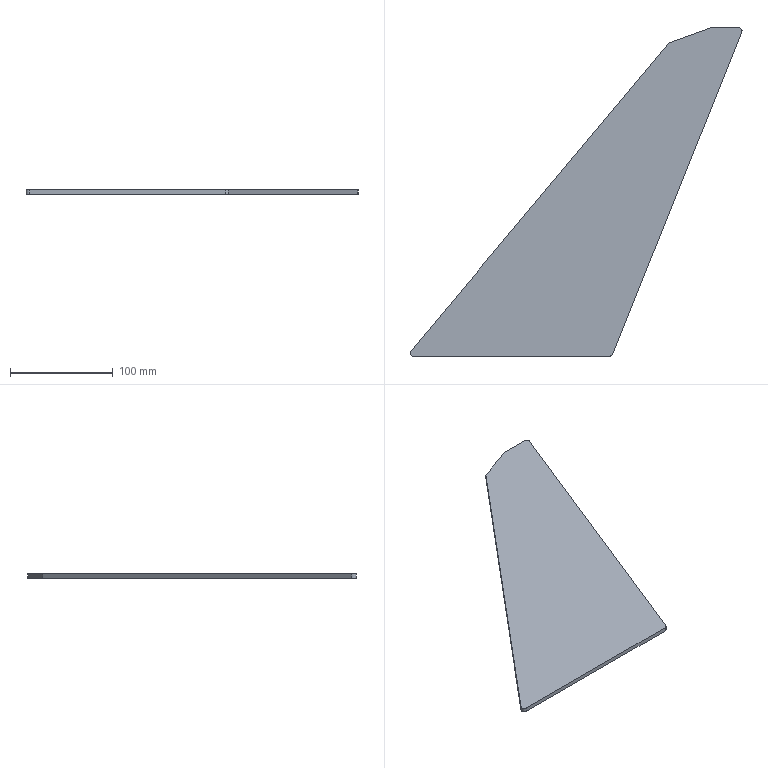Component | SolidWorks | 03-01MotorBracket1-1 | 1 solid | 11 faces | box 323.64 x 320 x 4 mm | volume 165534 mm3 | plane 7 | cylinder 4 | commonest cylinder face diameters 6 x4
STEP:
#1=COLOUR_RGB('',0.7922,0.8196,0.9333);
#2=FILL_AREA_STYLE_COLOUR('',#1);
#3=FILL_AREA_STYLE('',(#2));
#4=SURFACE_STYLE_FILL_AREA(#3);
#5=SURFACE_SIDE_STYLE('',(#4));
#6=SURFACE_STYLE_USAGE(.BOTH.,#5);
#7=PRESENTATION_STYLE_ASSIGNMENT((#6));
#8=CARTESIAN_POINT('',(11.927,12.48,14.961));
#9=VERTEX_POINT('',#8);
#10=CARTESIAN_POINT('',(11.918,12.436,14.961));
#11=VERTEX_POINT('',#10);
#12=CARTESIAN_POINT('',(11.809,12.48,14.961));
#13=DIRECTION('',(0.,0.,-1.));
#14=DIRECTION('',(1.,0.,0.));
#15=AXIS2_PLACEMENT_3D('',#12,#13,#14);
#16=CIRCLE('',#15,0.1181);
#17=EDGE_CURVE('',#9,#11,#16,.T.);
#18=ORIENTED_EDGE('',*,*,#17,.F.);
#19=CARTESIAN_POINT('',(11.927,12.48,15.118));
#20=VERTEX_POINT('',#19);
#21=CARTESIAN_POINT('',(11.927,12.48,14.961));
#22=DIRECTION('',(0.,0.,1.));
#23=VECTOR('',#22,39.37);
#24=LINE('',#21,#23);
#25=EDGE_CURVE('',#9,#20,#24,.T.);
#26=ORIENTED_EDGE('',*,*,#25,.T.);
#27=CARTESIAN_POINT('',(11.918,12.436,15.118));
#28=VERTEX_POINT('',#27);
#29=CARTESIAN_POINT('',(11.809,12.48,15.118));
#30=DIRECTION('',(0.,0.,1.));
#31=DIRECTION('',(1.,0.,0.));
#32=AXIS2_PLACEMENT_3D('',#29,#30,#31);
#33=CIRCLE('',#32,0.1181);
#34=EDGE_CURVE('',#28,#20,#33,.T.);
#35=ORIENTED_EDGE('',*,*,#34,.F.);
#36=CARTESIAN_POINT('',(11.918,12.436,14.961));
#37=DIRECTION('',(0.,0.,1.));
#38=VECTOR('',#37,39.37);
#39=LINE('',#36,#38);
#40=EDGE_CURVE('',#11,#28,#39,.T.);
#41=ORIENTED_EDGE('',*,*,#40,.F.);
#42=EDGE_LOOP('',(#18,#26,#35,#41));
#43=FACE_OUTER_BOUND('',#42,.T.);
#44=CARTESIAN_POINT('',(11.809,12.48,14.961));
#45=DIRECTION('',(0.,0.,1.));
#46=DIRECTION('',(1.,0.,0.));
#47=AXIS2_PLACEMENT_3D('',#44,#45,#46);
#48=CYLINDRICAL_SURFACE('',#47,0.1181);
#49=ADVANCED_FACE('',(#43),#48,.T.);
#50=CARTESIAN_POINT('',(9.14,12.025,15.118));
#51=VERTEX_POINT('',#50);
#52=CARTESIAN_POINT('',(-0.7874,0.194,15.118));
#53=VERTEX_POINT('',#52);
#54=CARTESIAN_POINT('',(9.621,12.598,15.118));
#55=DIRECTION('',(-0.6428,-0.766,0.));
#56=VECTOR('',#55,39.37);
#57=LINE('',#54,#56);
#58=EDGE_CURVE('',#51,#53,#57,.T.);
#59=ORIENTED_EDGE('',*,*,#58,.F.);
#60=CARTESIAN_POINT('',(9.14,12.025,14.961));
#61=VERTEX_POINT('',#60);
#62=CARTESIAN_POINT('',(9.14,12.025,14.724));
#63=DIRECTION('',(0.,0.,1.));
#64=VECTOR('',#63,39.37);
#65=LINE('',#62,#64);
#66=EDGE_CURVE('',#61,#51,#65,.T.);
#67=ORIENTED_EDGE('',*,*,#66,.F.);
#68=CARTESIAN_POINT('',(-0.7874,0.194,14.961));
#69=VERTEX_POINT('',#68);
#70=CARTESIAN_POINT('',(9.621,12.598,14.961));
#71=DIRECTION('',(-0.6428,-0.766,0.));
#72=VECTOR('',#71,39.37);
#73=LINE('',#70,#72);
#74=EDGE_CURVE('',#61,#69,#73,.T.);
#75=ORIENTED_EDGE('',*,*,#74,.T.);
#76=CARTESIAN_POINT('',(-0.7874,0.194,14.961));
#77=DIRECTION('',(0.,0.,1.));
#78=VECTOR('',#77,39.37);
#79=LINE('',#76,#78);
#80=EDGE_CURVE('',#69,#53,#79,.T.);
#81=ORIENTED_EDGE('',*,*,#80,.T.);
#82=EDGE_LOOP('',(#59,#67,#75,#81));
#83=FACE_OUTER_BOUND('',#82,.T.);
#84=CARTESIAN_POINT('',(9.621,12.598,14.961));
#85=DIRECTION('',(-0.766,0.6428,0.));
#86=DIRECTION('',(-0.6428,-0.766,0.));
#87=AXIS2_PLACEMENT_3D('',#84,#85,#86);
#88=PLANE('',#87);
#89=ADVANCED_FACE('',(#83),#88,.T.);
#90=CARTESIAN_POINT('',(11.809,12.598,14.961));
#91=VERTEX_POINT('',#90);
#92=CARTESIAN_POINT('',(10.715,12.598,14.961));
#93=VERTEX_POINT('',#92);
#94=CARTESIAN_POINT('',(11.983,12.598,14.961));
#95=DIRECTION('',(-1.,-0.,0.));
#96=VECTOR('',#95,39.37);
#97=LINE('',#94,#96);
#98=EDGE_CURVE('',#91,#93,#97,.T.);
#99=ORIENTED_EDGE('',*,*,#98,.T.);
#100=CARTESIAN_POINT('',(10.715,12.598,15.118));
#101=VERTEX_POINT('',#100);
#102=CARTESIAN_POINT('',(10.715,12.598,14.724));
#103=DIRECTION('',(0.,0.,1.));
#104=VECTOR('',#103,39.37);
#105=LINE('',#102,#104);
#106=EDGE_CURVE('',#93,#101,#105,.T.);
#107=ORIENTED_EDGE('',*,*,#106,.T.);
#108=CARTESIAN_POINT('',(11.809,12.598,15.118));
#109=VERTEX_POINT('',#108);
#110=CARTESIAN_POINT('',(11.983,12.598,15.118));
#111=DIRECTION('',(-1.,-0.,0.));
#112=VECTOR('',#111,39.37);
#113=LINE('',#110,#112);
#114=EDGE_CURVE('',#109,#101,#113,.T.);
#115=ORIENTED_EDGE('',*,*,#114,.F.);
#116=CARTESIAN_POINT('',(11.809,12.598,14.961));
#117=DIRECTION('',(0.,0.,-1.));
#118=VECTOR('',#117,39.37);
#119=LINE('',#116,#118);
#120=EDGE_CURVE('',#109,#91,#119,.T.);
#121=ORIENTED_EDGE('',*,*,#120,.T.);
#122=EDGE_LOOP('',(#99,#107,#115,#121));
#123=FACE_OUTER_BOUND('',#122,.T.);
#124=CARTESIAN_POINT('',(11.983,12.598,14.961));
#125=DIRECTION('',(-0.,1.,0.));
#126=DIRECTION('',(-1.,-0.,0.));
#127=AXIS2_PLACEMENT_3D('',#124,#125,#126);
#128=PLANE('',#127);
#129=ADVANCED_FACE('',(#123),#128,.T.);
#130=CARTESIAN_POINT('',(-3.635,7.376,14.961));
#131=DIRECTION('',(-0.9397,-0.342,0.));
#132=VECTOR('',#131,39.37);
#133=LINE('',#130,#132);
#134=EDGE_CURVE('',#93,#61,#133,.T.);
#135=ORIENTED_EDGE('',*,*,#134,.F.);
#136=ORIENTED_EDGE('',*,*,#98,.F.);
#137=CARTESIAN_POINT('',(11.809,12.48,14.961));
#138=DIRECTION('',(0.,0.,-1.));
#139=DIRECTION('',(1.,0.,0.));
#140=AXIS2_PLACEMENT_3D('',#137,#138,#139);
#141=CIRCLE('',#140,0.1181);
#142=EDGE_CURVE('',#91,#9,#141,.T.);
#143=ORIENTED_EDGE('',*,*,#142,.T.);
#144=ORIENTED_EDGE('',*,*,#17,.T.);
#145=CARTESIAN_POINT('',(6.954,0.07409,14.961));
#146=VERTEX_POINT('',#145);
#147=CARTESIAN_POINT('',(6.924,-0.,14.961));
#148=DIRECTION('',(0.3727,0.928,0.));
#149=VECTOR('',#148,39.37);
#150=LINE('',#147,#149);
#151=EDGE_CURVE('',#146,#11,#150,.T.);
#152=ORIENTED_EDGE('',*,*,#151,.F.);
#153=CARTESIAN_POINT('',(6.844,-0.,14.961));
#154=VERTEX_POINT('',#153);
#155=CARTESIAN_POINT('',(6.844,0.1181,14.961));
#156=DIRECTION('',(0.,0.,-1.));
#157=DIRECTION('',(1.,-0.,0.));
#158=AXIS2_PLACEMENT_3D('',#155,#156,#157);
#159=CIRCLE('',#158,0.1181);
#160=EDGE_CURVE('',#146,#154,#159,.T.);
#161=ORIENTED_EDGE('',*,*,#160,.T.);
#162=CARTESIAN_POINT('',(-0.6969,-0.,14.961));
#163=VERTEX_POINT('',#162);
#164=CARTESIAN_POINT('',(-0.9502,-0.,14.961));
#165=DIRECTION('',(1.,0.,0.));
#166=VECTOR('',#165,39.37);
#167=LINE('',#164,#166);
#168=EDGE_CURVE('',#163,#154,#167,.T.);
#169=ORIENTED_EDGE('',*,*,#168,.F.);
#170=CARTESIAN_POINT('',(-0.6969,0.1181,14.961));
#171=DIRECTION('',(0.,0.,-1.));
#172=DIRECTION('',(1.,0.,0.));
#173=AXIS2_PLACEMENT_3D('',#170,#171,#172);
#174=CIRCLE('',#173,0.1181);
#175=EDGE_CURVE('',#163,#69,#174,.T.);
#176=ORIENTED_EDGE('',*,*,#175,.T.);
#177=ORIENTED_EDGE('',*,*,#74,.F.);
#178=EDGE_LOOP('',(#135,#136,#143,#144,#152,#161,#169,#176,#177));
#179=FACE_OUTER_BOUND('',#178,.T.);
#180=CARTESIAN_POINT('',(-0.9502,-0.,14.961));
#181=DIRECTION('',(0.,0.,1.));
#182=DIRECTION('',(1.,0.,0.));
#183=AXIS2_PLACEMENT_3D('',#180,#181,#182);
#184=PLANE('',#183);
#185=ADVANCED_FACE('',(#179),#184,.F.);
#186=ORIENTED_EDGE('',*,*,#114,.T.);
#187=CARTESIAN_POINT('',(-3.635,7.376,15.118));
#188=DIRECTION('',(-0.9397,-0.342,0.));
#189=VECTOR('',#188,39.37);
#190=LINE('',#187,#189);
#191=EDGE_CURVE('',#101,#51,#190,.T.);
#192=ORIENTED_EDGE('',*,*,#191,.T.);
#193=ORIENTED_EDGE('',*,*,#58,.T.);
#194=CARTESIAN_POINT('',(-0.6969,-0.,15.118));
#195=VERTEX_POINT('',#194);
#196=CARTESIAN_POINT('',(-0.6969,0.1181,15.118));
#197=DIRECTION('',(0.,0.,1.));
#198=DIRECTION('',(1.,0.,0.));
#199=AXIS2_PLACEMENT_3D('',#196,#197,#198);
#200=CIRCLE('',#199,0.1181);
#201=EDGE_CURVE('',#53,#195,#200,.T.);
#202=ORIENTED_EDGE('',*,*,#201,.T.);
#203=CARTESIAN_POINT('',(6.844,-0.,15.118));
#204=VERTEX_POINT('',#203);
#205=CARTESIAN_POINT('',(-0.9502,-0.,15.118));
#206=DIRECTION('',(1.,0.,0.));
#207=VECTOR('',#206,39.37);
#208=LINE('',#205,#207);
#209=EDGE_CURVE('',#195,#204,#208,.T.);
#210=ORIENTED_EDGE('',*,*,#209,.T.);
#211=CARTESIAN_POINT('',(6.954,0.07409,15.118));
#212=VERTEX_POINT('',#211);
#213=CARTESIAN_POINT('',(6.844,0.1181,15.118));
#214=DIRECTION('',(0.,0.,1.));
#215=DIRECTION('',(1.,0.,0.));
#216=AXIS2_PLACEMENT_3D('',#213,#214,#215);
#217=CIRCLE('',#216,0.1181);
#218=EDGE_CURVE('',#204,#212,#217,.T.);
#219=ORIENTED_EDGE('',*,*,#218,.T.);
#220=CARTESIAN_POINT('',(6.924,-0.,15.118));
#221=DIRECTION('',(0.3727,0.928,0.));
#222=VECTOR('',#221,39.37);
#223=LINE('',#220,#222);
#224=EDGE_CURVE('',#212,#28,#223,.T.);
#225=ORIENTED_EDGE('',*,*,#224,.T.);
#226=ORIENTED_EDGE('',*,*,#34,.T.);
#227=CARTESIAN_POINT('',(11.809,12.48,15.118));
#228=DIRECTION('',(0.,0.,1.));
#229=DIRECTION('',(1.,0.,0.));
#230=AXIS2_PLACEMENT_3D('',#227,#228,#229);
#231=CIRCLE('',#230,0.1181);
#232=EDGE_CURVE('',#20,#109,#231,.T.);
#233=ORIENTED_EDGE('',*,*,#232,.T.);
#234=EDGE_LOOP('',(#186,#192,#193,#202,#210,#219,#225,#226,#233));
#235=FACE_OUTER_BOUND('',#234,.T.);
#236=CARTESIAN_POINT('',(-0.9502,-0.,15.118));
#237=DIRECTION('',(0.,0.,1.));
#238=DIRECTION('',(1.,0.,0.));
#239=AXIS2_PLACEMENT_3D('',#236,#237,#238);
#240=PLANE('',#239);
#241=ADVANCED_FACE('',(#235),#240,.T.);
#242=ORIENTED_EDGE('',*,*,#224,.F.);
#243=CARTESIAN_POINT('',(6.954,0.07409,14.961));
#244=DIRECTION('',(0.,0.,-1.));
#245=VECTOR('',#244,39.37);
#246=LINE('',#243,#245);
#247=EDGE_CURVE('',#212,#146,#246,.T.);
#248=ORIENTED_EDGE('',*,*,#247,.T.);
#249=ORIENTED_EDGE('',*,*,#151,.T.);
#250=ORIENTED_EDGE('',*,*,#40,.T.);
#251=EDGE_LOOP('',(#242,#248,#249,#250));
#252=FACE_OUTER_BOUND('',#251,.T.);
#253=CARTESIAN_POINT('',(6.924,-0.,14.961));
#254=DIRECTION('',(0.928,-0.3727,0.));
#255=DIRECTION('',(0.3727,0.928,0.));
#256=AXIS2_PLACEMENT_3D('',#253,#254,#255);
#257=PLANE('',#256);
#258=ADVANCED_FACE('',(#252),#257,.T.);
#259=ORIENTED_EDGE('',*,*,#168,.T.);
#260=CARTESIAN_POINT('',(6.844,-0.,14.961));
#261=DIRECTION('',(0.,0.,1.));
#262=VECTOR('',#261,39.37);
#263=LINE('',#260,#262);
#264=EDGE_CURVE('',#154,#204,#263,.T.);
#265=ORIENTED_EDGE('',*,*,#264,.T.);
#266=ORIENTED_EDGE('',*,*,#209,.F.);
#267=CARTESIAN_POINT('',(-0.6969,-0.,14.961));
#268=DIRECTION('',(0.,0.,-1.));
#269=VECTOR('',#268,39.37);
#270=LINE('',#267,#269);
#271=EDGE_CURVE('',#195,#163,#270,.T.);
#272=ORIENTED_EDGE('',*,*,#271,.T.);
#273=EDGE_LOOP('',(#259,#265,#266,#272));
#274=FACE_OUTER_BOUND('',#273,.T.);
#275=CARTESIAN_POINT('',(-0.9502,-0.,14.961));
#276=DIRECTION('',(0.,-1.,0.));
#277=DIRECTION('',(0.,0.,-1.));
#278=AXIS2_PLACEMENT_3D('',#275,#276,#277);
#279=PLANE('',#278);
#280=ADVANCED_FACE('',(#274),#279,.T.);
#281=ORIENTED_EDGE('',*,*,#160,.F.);
#282=ORIENTED_EDGE('',*,*,#247,.F.);
#283=ORIENTED_EDGE('',*,*,#218,.F.);
#284=ORIENTED_EDGE('',*,*,#264,.F.);
#285=EDGE_LOOP('',(#281,#282,#283,#284));
#286=FACE_OUTER_BOUND('',#285,.T.);
#287=CARTESIAN_POINT('',(6.844,0.1181,14.961));
#288=DIRECTION('',(0.,0.,1.));
#289=DIRECTION('',(1.,0.,0.));
#290=AXIS2_PLACEMENT_3D('',#287,#288,#289);
#291=CYLINDRICAL_SURFACE('',#290,0.1181);
#292=ADVANCED_FACE('',(#286),#291,.T.);
#293=ORIENTED_EDGE('',*,*,#175,.F.);
#294=ORIENTED_EDGE('',*,*,#271,.F.);
#295=ORIENTED_EDGE('',*,*,#201,.F.);
#296=ORIENTED_EDGE('',*,*,#80,.F.);
#297=EDGE_LOOP('',(#293,#294,#295,#296));
#298=FACE_OUTER_BOUND('',#297,.T.);
#299=CARTESIAN_POINT('',(-0.6969,0.1181,14.961));
#300=DIRECTION('',(0.,0.,1.));
#301=DIRECTION('',(1.,0.,0.));
#302=AXIS2_PLACEMENT_3D('',#299,#300,#301);
#303=CYLINDRICAL_SURFACE('',#302,0.1181);
#304=ADVANCED_FACE('',(#298),#303,.T.);
#305=ORIENTED_EDGE('',*,*,#25,.F.);
#306=ORIENTED_EDGE('',*,*,#142,.F.);
#307=ORIENTED_EDGE('',*,*,#120,.F.);
#308=ORIENTED_EDGE('',*,*,#232,.F.);
#309=EDGE_LOOP('',(#305,#306,#307,#308));
#310=FACE_OUTER_BOUND('',#309,.T.);
#311=CARTESIAN_POINT('',(11.809,12.48,14.961));
#312=DIRECTION('',(0.,0.,1.));
#313=DIRECTION('',(1.,0.,0.));
#314=AXIS2_PLACEMENT_3D('',#311,#312,#313);
#315=CYLINDRICAL_SURFACE('',#314,0.1181);
#316=ADVANCED_FACE('',(#310),#315,.T.);
#317=ORIENTED_EDGE('',*,*,#134,.T.);
#318=ORIENTED_EDGE('',*,*,#66,.T.);
#319=ORIENTED_EDGE('',*,*,#191,.F.);
#320=ORIENTED_EDGE('',*,*,#106,.F.);
#321=EDGE_LOOP('',(#317,#318,#319,#320));
#322=FACE_OUTER_BOUND('',#321,.T.);
#323=CARTESIAN_POINT('',(-3.635,7.376,14.724));
#324=DIRECTION('',(-0.342,0.9397,0.));
#325=DIRECTION('',(-0.9397,-0.342,0.));
#326=AXIS2_PLACEMENT_3D('',#323,#324,#325);
#327=PLANE('',#326);
#328=ADVANCED_FACE('',(#322),#327,.T.);
#329=CLOSED_SHELL('',(#49,#89,#129,#185,#241,#258,#280,#292,#304,#316,#328));
#330=MANIFOLD_SOLID_BREP('',#329);
#331=STYLED_ITEM('',(#7),#330);
#332=(LENGTH_UNIT()NAMED_UNIT(*)SI_UNIT($,.METRE.));
#333=LENGTH_MEASURE_WITH_UNIT(LENGTH_MEASURE(0.0254),#332);
#334=DIMENSIONAL_EXPONENTS(1.,0.,0.,0.,0.,0.,0.);
#335=(CONVERSION_BASED_UNIT('',#333)LENGTH_UNIT()NAMED_UNIT(#334));
#336=UNCERTAINTY_MEASURE_WITH_UNIT(LENGTH_MEASURE(0.00001),#335,'','');
#337=(NAMED_UNIT(*)PLANE_ANGLE_UNIT()SI_UNIT($,.RADIAN.));
#338=(NAMED_UNIT(*)SI_UNIT($,.STERADIAN.)SOLID_ANGLE_UNIT());
#339=(GEOMETRIC_REPRESENTATION_CONTEXT(3)GLOBAL_UNCERTAINTY_ASSIGNED_CONTEXT((#336))GLOBAL_UNIT_ASSIGNED_CONTEXT((#335,#337,#338))REPRESENTATION_CONTEXT('',''));
#340=MECHANICAL_DESIGN_GEOMETRIC_PRESENTATION_REPRESENTATION('',(#331),#339);
#341=CARTESIAN_POINT('',(0.,0.,0.));
#342=DIRECTION('',(0.,0.,1.));
#343=DIRECTION('',(1.,0.,0.));
#344=AXIS2_PLACEMENT_3D('',#341,#342,#343);
#345=(LENGTH_UNIT()NAMED_UNIT(*)SI_UNIT($,.METRE.));
#346=LENGTH_MEASURE_WITH_UNIT(LENGTH_MEASURE(0.0254),#345);
#347=DIMENSIONAL_EXPONENTS(1.,0.,0.,0.,0.,0.,0.);
#348=(CONVERSION_BASED_UNIT('',#346)LENGTH_UNIT()NAMED_UNIT(#347));
#349=UNCERTAINTY_MEASURE_WITH_UNIT(LENGTH_MEASURE(0.00001),#348,'','');
#350=(NAMED_UNIT(*)PLANE_ANGLE_UNIT()SI_UNIT($,.RADIAN.));
#351=(NAMED_UNIT(*)SI_UNIT($,.STERADIAN.)SOLID_ANGLE_UNIT());
#352=(GEOMETRIC_REPRESENTATION_CONTEXT(3)GLOBAL_UNCERTAINTY_ASSIGNED_CONTEXT((#349))GLOBAL_UNIT_ASSIGNED_CONTEXT((#348,#350,#351))REPRESENTATION_CONTEXT('',''));
#353=ADVANCED_BREP_SHAPE_REPRESENTATION('',(#330,#344),#352);
#354=PRESENTATION_LAYER_ASSIGNMENT('','',(#331));